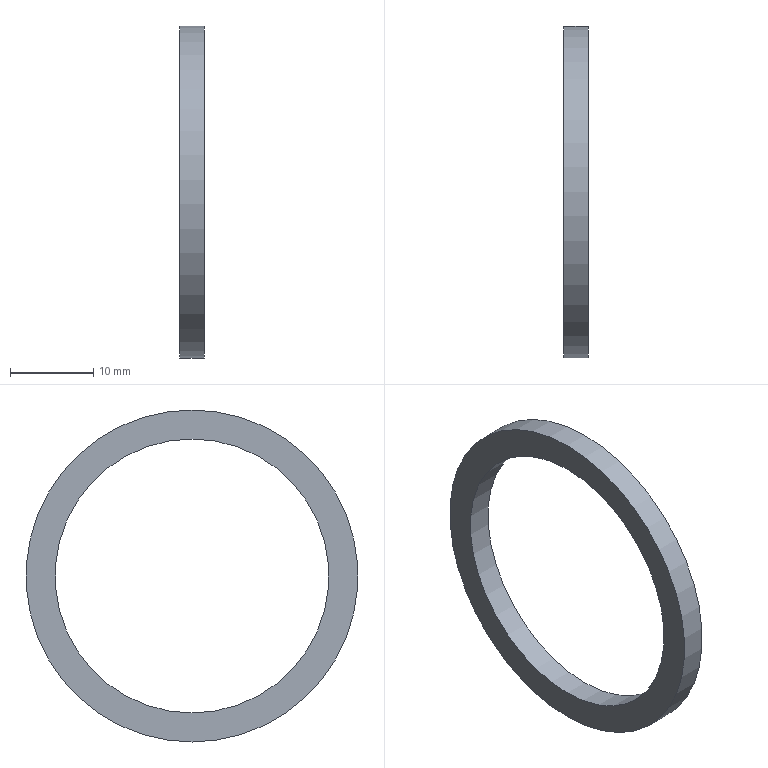Component | NX | SEAL_RING | 1 solid | 4 faces | box 3 x 40 x 40 mm | volume 1204 mm3 | plane 2 | cylinder 2 | commonest cylinder face diameters 33 x1 40 x1
STEP:
#1=CARTESIAN_POINT('',(0.,0.,0.));
#2=DIRECTION('',(0.,0.,1.));
#3=DIRECTION('',(1.,0.,0.));
#4=AXIS2_PLACEMENT_3D('',#1,#2,#3);
#5=CARTESIAN_POINT('',(106.5,0.,-16.5));
#6=VERTEX_POINT('',#5);
#7=CARTESIAN_POINT('',(106.5,0.,0.));
#8=DIRECTION('',(1.,0.,0.));
#9=DIRECTION('',(0.,0.,-1.));
#10=AXIS2_PLACEMENT_3D('',#7,#8,#9);
#11=CIRCLE('',#10,16.5);
#12=CARTESIAN_POINT('',(106.5,0.,20.));
#13=DIRECTION('',(-1.,0.,0.));
#14=DIRECTION('',(0.,0.,1.));
#15=AXIS2_PLACEMENT_3D('',#12,#13,#14);
#16=PLANE('',#15);
#17=CARTESIAN_POINT('',(-36.5,0.));
#18=CARTESIAN_POINT('',(-36.5,28.579));
#19=CARTESIAN_POINT('',(-11.75,14.289));
#20=CARTESIAN_POINT('',(13.,0.));
#21=CARTESIAN_POINT('',(-11.75,-14.289));
#22=CARTESIAN_POINT('',(-36.5,-28.579));
#23=CARTESIAN_POINT('',(-36.5,0.));
#24=(BOUNDED_CURVE()B_SPLINE_CURVE(2,(#17,#18,#19,#20,#21,#22,#23),.UNSPECIFIED.,.T.,.F.)B_SPLINE_CURVE_WITH_KNOTS((1,2,2,2,2,1),(-2.094,0.,2.094,4.189,6.283,8.378),.UNSPECIFIED.)CURVE()GEOMETRIC_REPRESENTATION_ITEM()RATIONAL_B_SPLINE_CURVE((1.,0.5,1.,0.5,1.,0.5,1.))REPRESENTATION_ITEM(''));
#25=(GEOMETRIC_REPRESENTATION_CONTEXT(2)PARAMETRIC_REPRESENTATION_CONTEXT()REPRESENTATION_CONTEXT('',''));
#26=DEFINITIONAL_REPRESENTATION('',(#24),#25);
#27=PCURVE('',#16,#26);
#28=CARTESIAN_POINT('',(103.5,0.,0.));
#29=DIRECTION('',(1.,0.,0.));
#30=DIRECTION('',(0.,0.,-1.));
#31=AXIS2_PLACEMENT_3D('',#28,#29,#30);
#32=CYLINDRICAL_SURFACE('',#31,16.5);
#33=CARTESIAN_POINT('',(0.,3.));
#34=DIRECTION('',(1.,0.));
#35=VECTOR('',#34,1.);
#36=LINE('',#33,#35);
#37=(GEOMETRIC_REPRESENTATION_CONTEXT(2)PARAMETRIC_REPRESENTATION_CONTEXT()REPRESENTATION_CONTEXT('',''));
#38=DEFINITIONAL_REPRESENTATION('',(#36),#37);
#39=PCURVE('',#32,#38);
#40=SURFACE_CURVE('',#11,(#27,#39),.PCURVE_S1.);
#41=EDGE_CURVE('',#6,#6,#40,.T.);
#42=ORIENTED_EDGE('',*,*,#41,.F.);
#43=EDGE_LOOP('',(#42));
#44=FACE_BOUND('',#43,.T.);
#45=CARTESIAN_POINT('',(106.5,0.,-20.));
#46=VERTEX_POINT('',#45);
#47=CARTESIAN_POINT('',(106.5,0.,0.));
#48=DIRECTION('',(1.,0.,0.));
#49=DIRECTION('',(0.,0.,-1.));
#50=AXIS2_PLACEMENT_3D('',#47,#48,#49);
#51=CIRCLE('',#50,20.);
#52=CARTESIAN_POINT('',(-40.,0.));
#53=CARTESIAN_POINT('',(-40.,34.641));
#54=CARTESIAN_POINT('',(-10.,17.321));
#55=CARTESIAN_POINT('',(20.,0.));
#56=CARTESIAN_POINT('',(-10.,-17.321));
#57=CARTESIAN_POINT('',(-40.,-34.641));
#58=CARTESIAN_POINT('',(-40.,0.));
#59=(BOUNDED_CURVE()B_SPLINE_CURVE(2,(#52,#53,#54,#55,#56,#57,#58),.UNSPECIFIED.,.T.,.F.)B_SPLINE_CURVE_WITH_KNOTS((1,2,2,2,2,1),(-2.094,0.,2.094,4.189,6.283,8.378),.UNSPECIFIED.)CURVE()GEOMETRIC_REPRESENTATION_ITEM()RATIONAL_B_SPLINE_CURVE((1.,0.5,1.,0.5,1.,0.5,1.))REPRESENTATION_ITEM(''));
#60=(GEOMETRIC_REPRESENTATION_CONTEXT(2)PARAMETRIC_REPRESENTATION_CONTEXT()REPRESENTATION_CONTEXT('',''));
#61=DEFINITIONAL_REPRESENTATION('',(#59),#60);
#62=PCURVE('',#16,#61);
#63=CARTESIAN_POINT('',(103.5,0.,0.));
#64=DIRECTION('',(1.,0.,0.));
#65=DIRECTION('',(0.,0.,-1.));
#66=AXIS2_PLACEMENT_3D('',#63,#64,#65);
#67=CYLINDRICAL_SURFACE('',#66,20.);
#68=CARTESIAN_POINT('',(0.,3.));
#69=DIRECTION('',(1.,0.));
#70=VECTOR('',#69,1.);
#71=LINE('',#68,#70);
#72=(GEOMETRIC_REPRESENTATION_CONTEXT(2)PARAMETRIC_REPRESENTATION_CONTEXT()REPRESENTATION_CONTEXT('',''));
#73=DEFINITIONAL_REPRESENTATION('',(#71),#72);
#74=PCURVE('',#67,#73);
#75=SURFACE_CURVE('',#51,(#62,#74),.PCURVE_S1.);
#76=EDGE_CURVE('',#46,#46,#75,.T.);
#77=ORIENTED_EDGE('',*,*,#76,.T.);
#78=EDGE_LOOP('',(#77));
#79=FACE_BOUND('',#78,.T.);
#80=ADVANCED_FACE('',(#44,#79),#16,.F.);
#81=CARTESIAN_POINT('',(103.5,0.,-16.5));
#82=VERTEX_POINT('',#81);
#83=CARTESIAN_POINT('',(103.5,0.,0.));
#84=DIRECTION('',(1.,0.,0.));
#85=DIRECTION('',(0.,0.,-1.));
#86=AXIS2_PLACEMENT_3D('',#83,#84,#85);
#87=CIRCLE('',#86,16.5);
#88=CARTESIAN_POINT('',(0.,0.));
#89=DIRECTION('',(1.,0.));
#90=VECTOR('',#89,1.);
#91=LINE('',#88,#90);
#92=(GEOMETRIC_REPRESENTATION_CONTEXT(2)PARAMETRIC_REPRESENTATION_CONTEXT()REPRESENTATION_CONTEXT('',''));
#93=DEFINITIONAL_REPRESENTATION('',(#91),#92);
#94=PCURVE('',#32,#93);
#95=CARTESIAN_POINT('',(103.5,0.,16.5));
#96=DIRECTION('',(1.,0.,0.));
#97=DIRECTION('',(0.,0.,-1.));
#98=AXIS2_PLACEMENT_3D('',#95,#96,#97);
#99=PLANE('',#98);
#100=CARTESIAN_POINT('',(16.5,0.));
#101=DIRECTION('',(1.,0.));
#102=AXIS2_PLACEMENT_2D('',#100,#101);
#103=CIRCLE('',#102,16.5);
#104=(GEOMETRIC_REPRESENTATION_CONTEXT(2)PARAMETRIC_REPRESENTATION_CONTEXT()REPRESENTATION_CONTEXT('',''));
#105=DEFINITIONAL_REPRESENTATION('',(#103),#104);
#106=PCURVE('',#99,#105);
#107=SURFACE_CURVE('',#87,(#94,#106),.PCURVE_S1.);
#108=EDGE_CURVE('',#82,#82,#107,.T.);
#109=ORIENTED_EDGE('',*,*,#108,.T.);
#110=CARTESIAN_POINT('',(103.5,0.,-16.5));
#111=CARTESIAN_POINT('',(106.5,0.,-16.5));
#112=B_SPLINE_CURVE_WITH_KNOTS('',1,(#110,#111),.UNSPECIFIED.,.F.,.F.,(2,2),(0.,3.),.PIECEWISE_BEZIER_KNOTS.);
#113=CARTESIAN_POINT('',(6.283,0.));
#114=DIRECTION('',(0.,1.));
#115=VECTOR('',#114,1.);
#116=LINE('',#113,#115);
#117=(GEOMETRIC_REPRESENTATION_CONTEXT(2)PARAMETRIC_REPRESENTATION_CONTEXT()REPRESENTATION_CONTEXT('',''));
#118=DEFINITIONAL_REPRESENTATION('',(#116),#117);
#119=PCURVE('',#32,#118);
#120=CARTESIAN_POINT('',(0.,0.));
#121=DIRECTION('',(0.,1.));
#122=VECTOR('',#121,1.);
#123=LINE('',#120,#122);
#124=(GEOMETRIC_REPRESENTATION_CONTEXT(2)PARAMETRIC_REPRESENTATION_CONTEXT()REPRESENTATION_CONTEXT('',''));
#125=DEFINITIONAL_REPRESENTATION('',(#123),#124);
#126=PCURVE('',#32,#125);
#127=SEAM_CURVE('',#112,(#119,#126),.PCURVE_S1.);
#128=EDGE_CURVE('',#82,#6,#127,.T.);
#129=ORIENTED_EDGE('',*,*,#128,.T.);
#130=ORIENTED_EDGE('',*,*,#41,.F.);
#131=ORIENTED_EDGE('',*,*,#128,.F.);
#132=EDGE_LOOP('',(#109,#129,#130,#131));
#133=FACE_BOUND('',#132,.F.);
#134=ADVANCED_FACE('',(#133),#32,.F.);
#135=CARTESIAN_POINT('',(103.5,0.,-20.));
#136=VERTEX_POINT('',#135);
#137=CARTESIAN_POINT('',(103.5,0.,0.));
#138=DIRECTION('',(1.,0.,0.));
#139=DIRECTION('',(0.,0.,-1.));
#140=AXIS2_PLACEMENT_3D('',#137,#138,#139);
#141=CIRCLE('',#140,20.);
#142=CARTESIAN_POINT('',(16.5,0.));
#143=DIRECTION('',(1.,0.));
#144=AXIS2_PLACEMENT_2D('',#142,#143);
#145=CIRCLE('',#144,20.);
#146=(GEOMETRIC_REPRESENTATION_CONTEXT(2)PARAMETRIC_REPRESENTATION_CONTEXT()REPRESENTATION_CONTEXT('',''));
#147=DEFINITIONAL_REPRESENTATION('',(#145),#146);
#148=PCURVE('',#99,#147);
#149=CARTESIAN_POINT('',(0.,0.));
#150=DIRECTION('',(1.,0.));
#151=VECTOR('',#150,1.);
#152=LINE('',#149,#151);
#153=(GEOMETRIC_REPRESENTATION_CONTEXT(2)PARAMETRIC_REPRESENTATION_CONTEXT()REPRESENTATION_CONTEXT('',''));
#154=DEFINITIONAL_REPRESENTATION('',(#152),#153);
#155=PCURVE('',#67,#154);
#156=SURFACE_CURVE('',#141,(#148,#155),.PCURVE_S1.);
#157=EDGE_CURVE('',#136,#136,#156,.T.);
#158=ORIENTED_EDGE('',*,*,#157,.F.);
#159=EDGE_LOOP('',(#158));
#160=FACE_BOUND('',#159,.T.);
#161=ORIENTED_EDGE('',*,*,#108,.T.);
#162=EDGE_LOOP('',(#161));
#163=FACE_BOUND('',#162,.T.);
#164=ADVANCED_FACE('',(#160,#163),#99,.F.);
#165=ORIENTED_EDGE('',*,*,#76,.F.);
#166=CARTESIAN_POINT('',(103.5,-0.,-20.));
#167=CARTESIAN_POINT('',(106.5,-0.,-20.));
#168=B_SPLINE_CURVE_WITH_KNOTS('',1,(#166,#167),.UNSPECIFIED.,.F.,.F.,(2,2),(0.,3.),.PIECEWISE_BEZIER_KNOTS.);
#169=CARTESIAN_POINT('',(0.,0.));
#170=DIRECTION('',(0.,1.));
#171=VECTOR('',#170,1.);
#172=LINE('',#169,#171);
#173=(GEOMETRIC_REPRESENTATION_CONTEXT(2)PARAMETRIC_REPRESENTATION_CONTEXT()REPRESENTATION_CONTEXT('',''));
#174=DEFINITIONAL_REPRESENTATION('',(#172),#173);
#175=PCURVE('',#67,#174);
#176=CARTESIAN_POINT('',(6.283,0.));
#177=DIRECTION('',(0.,1.));
#178=VECTOR('',#177,1.);
#179=LINE('',#176,#178);
#180=(GEOMETRIC_REPRESENTATION_CONTEXT(2)PARAMETRIC_REPRESENTATION_CONTEXT()REPRESENTATION_CONTEXT('',''));
#181=DEFINITIONAL_REPRESENTATION('',(#179),#180);
#182=PCURVE('',#67,#181);
#183=SEAM_CURVE('',#168,(#175,#182),.PCURVE_S1.);
#184=EDGE_CURVE('',#136,#46,#183,.T.);
#185=ORIENTED_EDGE('',*,*,#184,.F.);
#186=ORIENTED_EDGE('',*,*,#157,.T.);
#187=ORIENTED_EDGE('',*,*,#184,.T.);
#188=EDGE_LOOP('',(#165,#185,#186,#187));
#189=FACE_BOUND('',#188,.T.);
#190=ADVANCED_FACE('',(#189),#67,.T.);
#191=CLOSED_SHELL('',(#80,#134,#164,#190));
#192=MANIFOLD_SOLID_BREP('',#191);
#193=(LENGTH_UNIT()NAMED_UNIT(*)SI_UNIT(.MILLI.,.METRE.));
#194=UNCERTAINTY_MEASURE_WITH_UNIT(LENGTH_MEASURE(0.00001),#193,'','');
#195=(NAMED_UNIT(*)PLANE_ANGLE_UNIT()SI_UNIT($,.RADIAN.));
#196=(NAMED_UNIT(*)SI_UNIT($,.STERADIAN.)SOLID_ANGLE_UNIT());
#197=(GEOMETRIC_REPRESENTATION_CONTEXT(3)GLOBAL_UNCERTAINTY_ASSIGNED_CONTEXT((#194))GLOBAL_UNIT_ASSIGNED_CONTEXT((#193,#195,#196))REPRESENTATION_CONTEXT('',''));
#198=ADVANCED_BREP_SHAPE_REPRESENTATION('',(#4,#192),#197);